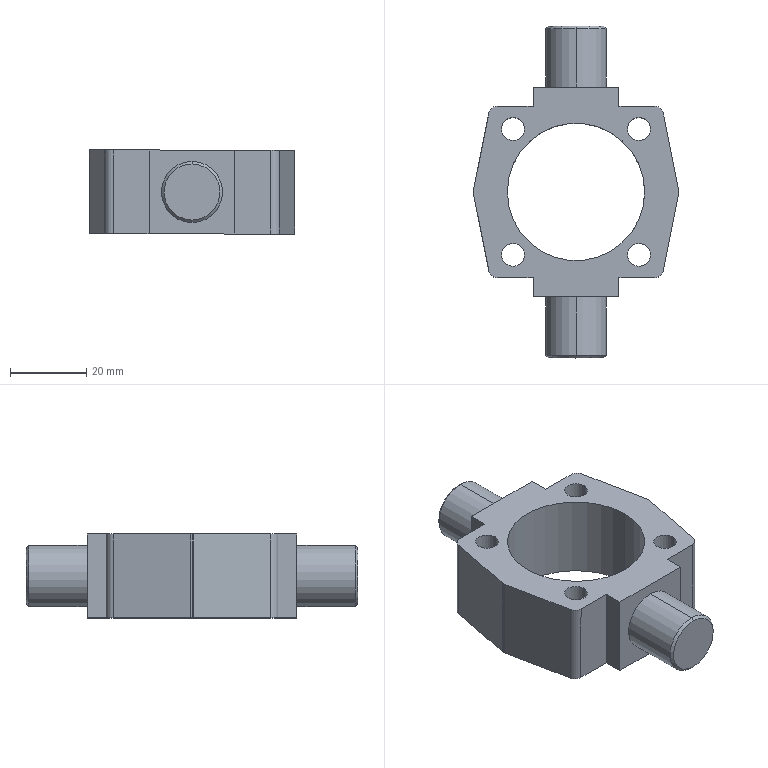Component | SolidWorks | RobotArmTelescopicCylinderSC32x500-1_MiddleEarFixingConnectionBlock-1 | 1 solid | 43 faces | box 53.93 x 87 x 22.06 mm | volume 35426 mm3 | cylinder 21 | plane 18 | cone 4 | commonest cylinder face diameters 6 x8 4.5 x7 16 x4 36 x2